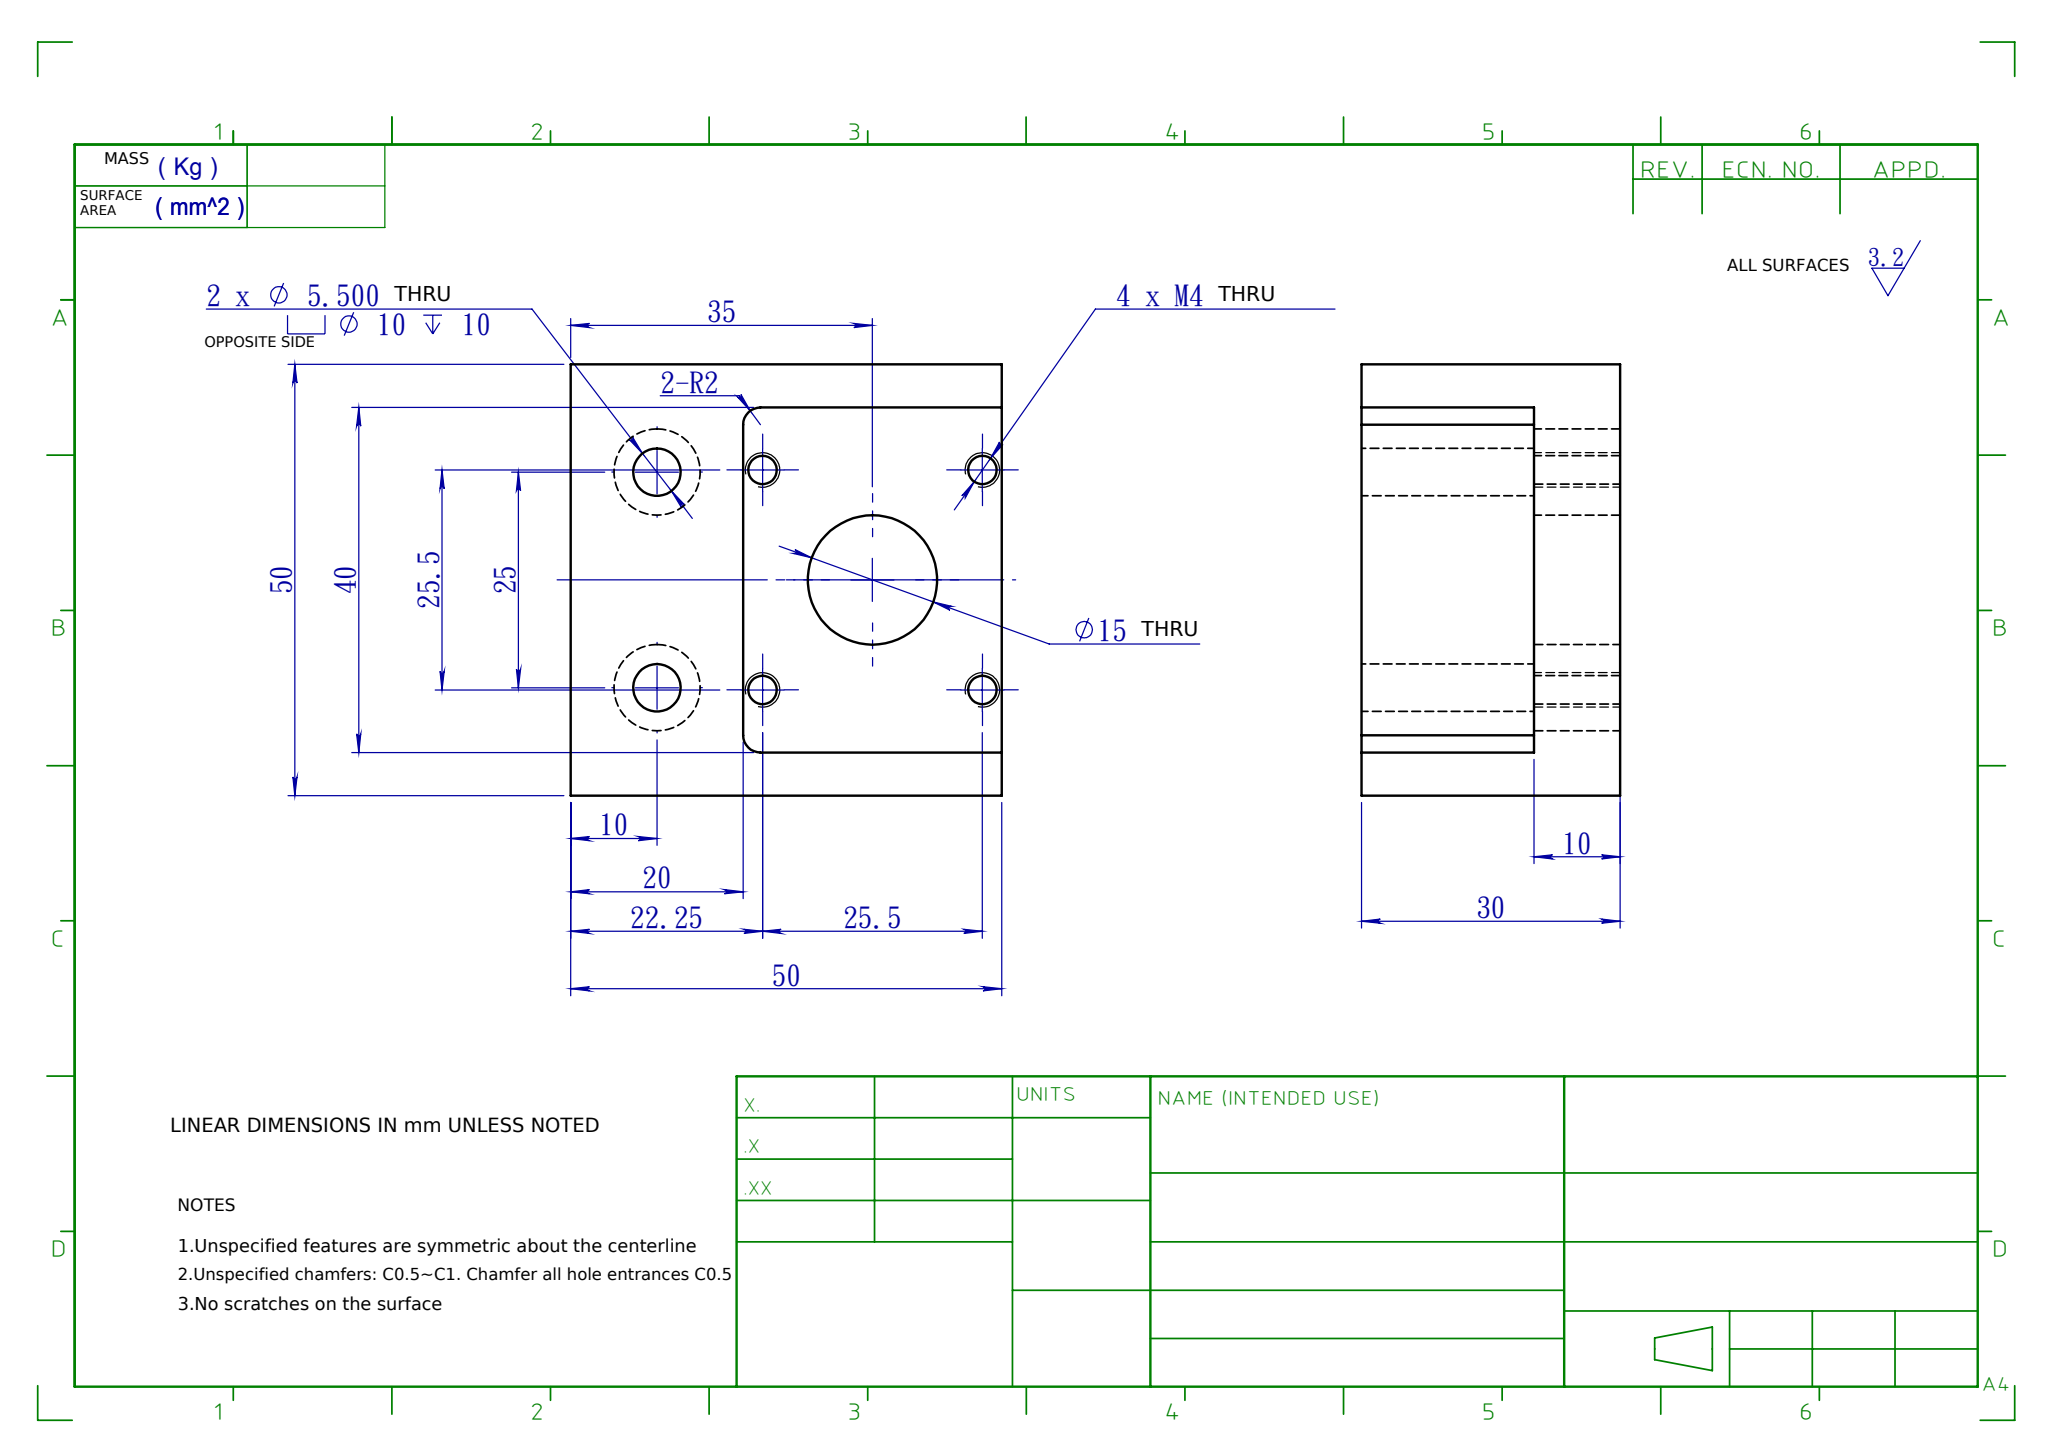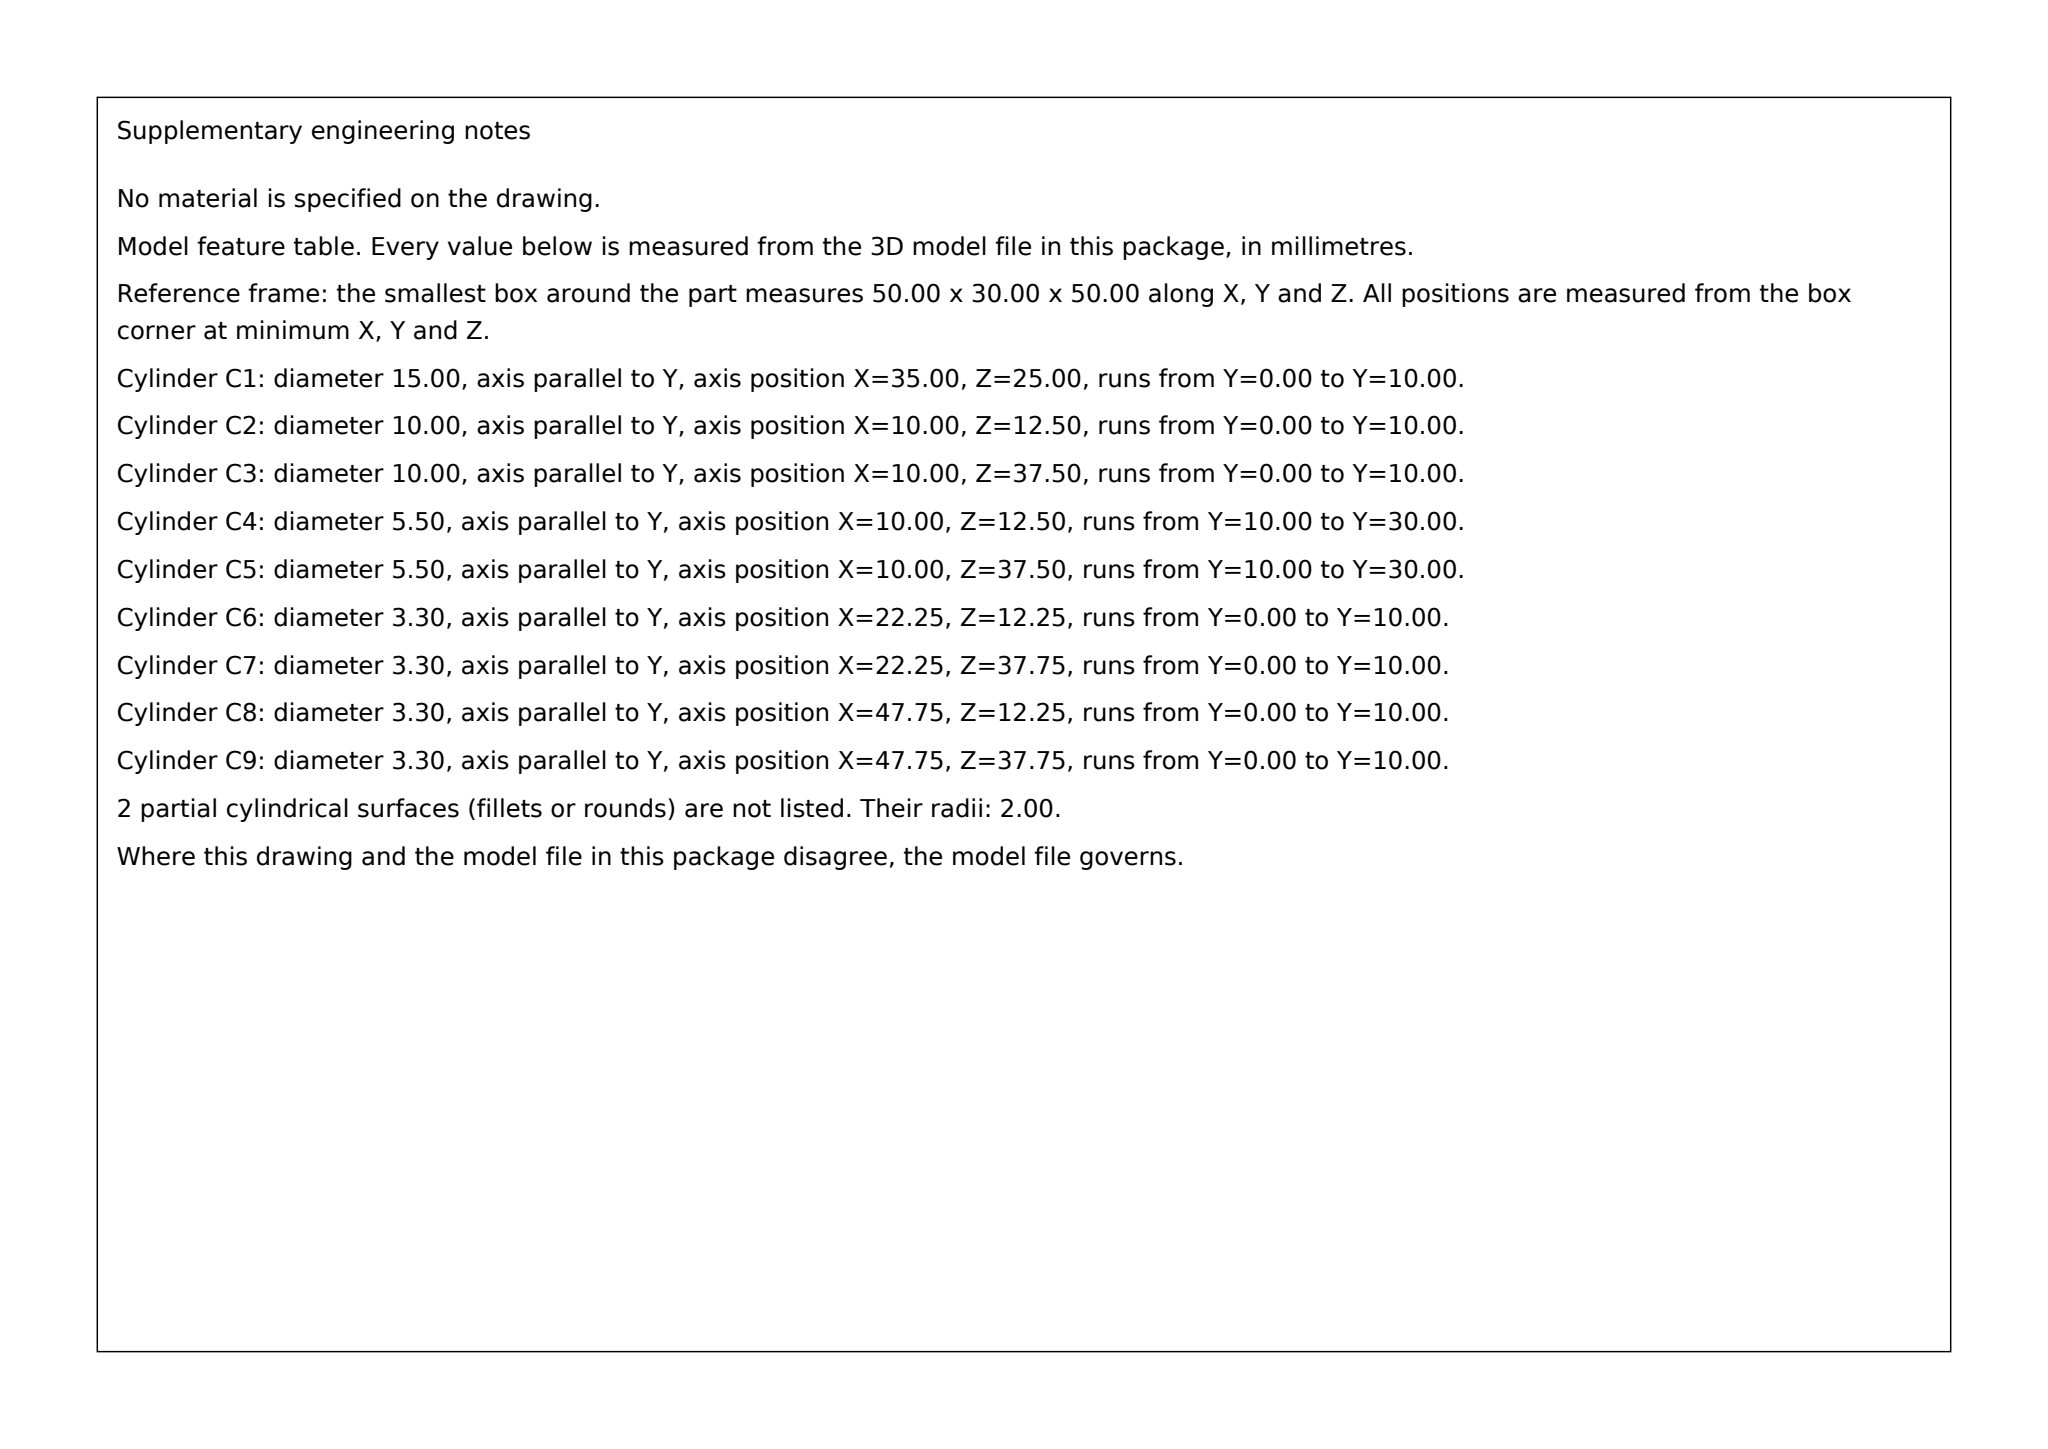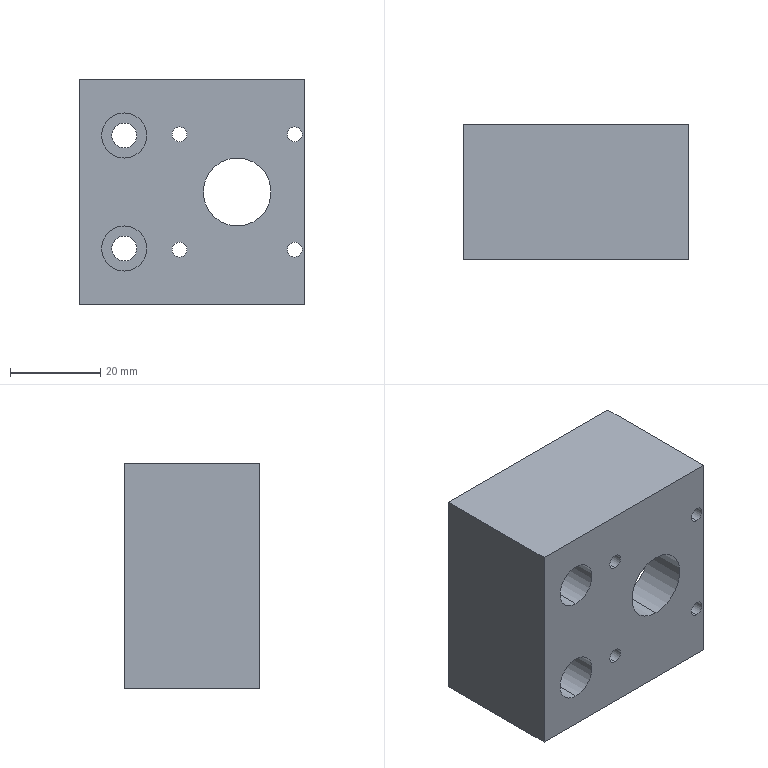Part | SolidWorks | mm | 1 solid | 32 faces | box 50 x 30 x 50 mm | volume 46404 mm3 | cylinder 20 | plane 12 | commonest cylinder face diameters 3.3 x8 10 x4 5.5 x4 15 x2 4 x2